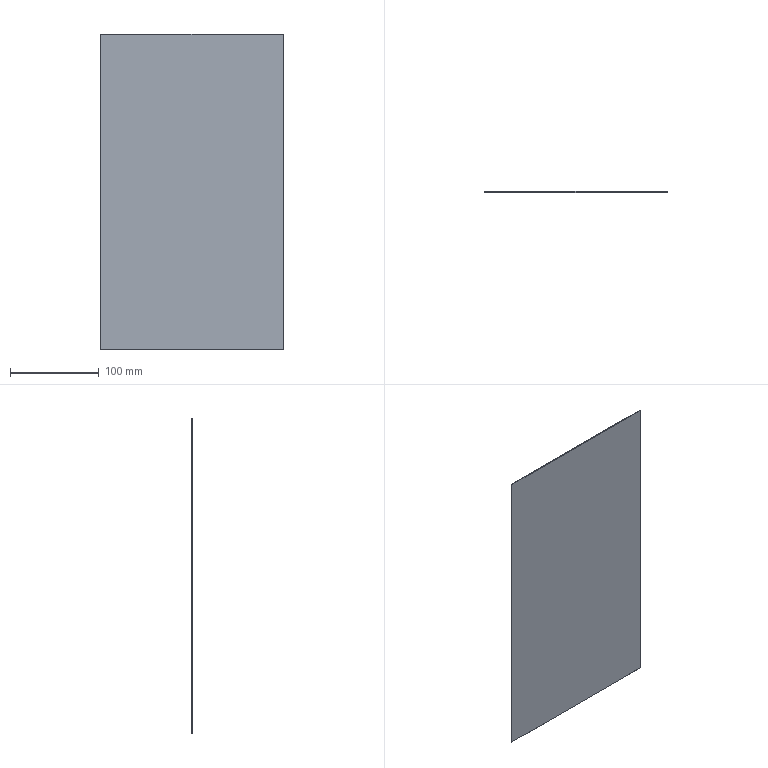Component | SolidWorks | SL021-1LGP-15.6.SL4PRT-1 | 1 solid | 6 faces | box 205 x 0.9 x 355 mm | volume 65498 mm3 | plane 6 | material AL6061
build123d program:
from build123d import *

# Parameters (mm, degrees)
SKETCH2_W           = 355
SKETCH2_H           = 205
BOSS_EXTRUDE1_DEPTH = 0.45


with BuildPart() as part:
    # Sketch2 → Boss-Extrude1 (new, symmetric)
    with BuildSketch(Plane(origin=(0, 0, 0), x_dir=(1, 0, 0), z_dir=(0, 1, 0))):
        Rectangle(SKETCH2_W, SKETCH2_H)
    extrude(amount=BOSS_EXTRUDE1_DEPTH, both=True)


solid = part.part

# Placed as in the assembly
solid = solid.moved(Location((-136.163, -149.949, -151.378), (0, 90, 0)))